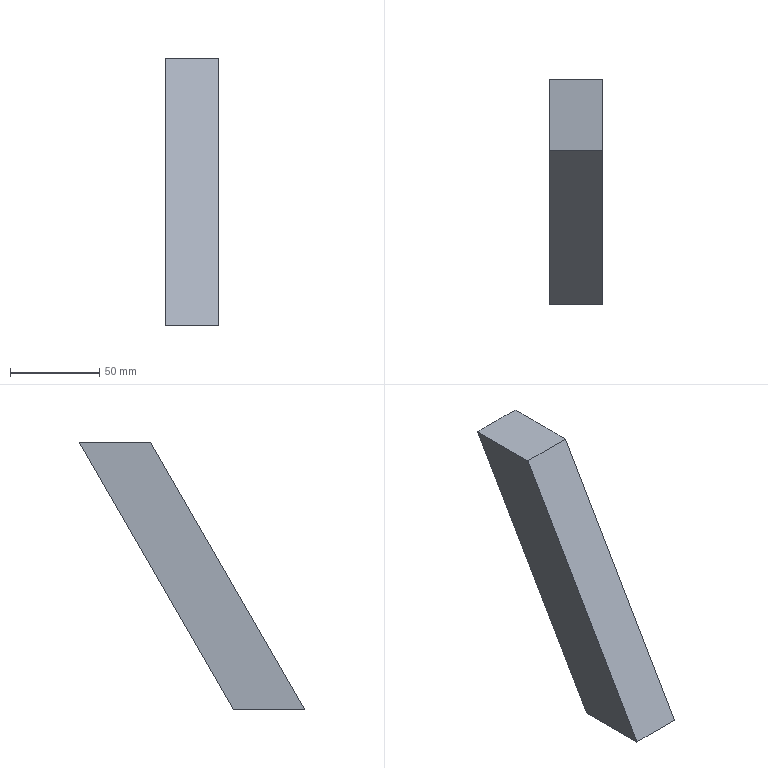Component | NX | AYAK_2 | 1 solid | 6 faces | box 30 x 126.6 x 150 mm | volume 180000 mm3 | plane 6
STEP:
#1=CARTESIAN_POINT('',(0.,0.,0.));
#2=DIRECTION('',(0.,0.,1.));
#3=DIRECTION('',(1.,0.,0.));
#4=AXIS2_PLACEMENT_3D('',#1,#2,#3);
#5=CARTESIAN_POINT('',(-1340.866,653.021,0.));
#6=VERTEX_POINT('',#5);
#7=CARTESIAN_POINT('',(-1340.866,693.021,0.));
#8=VERTEX_POINT('',#7);
#9=CARTESIAN_POINT('',(-1340.866,653.021,0.));
#10=DIRECTION('',(0.,1.,0.));
#11=VECTOR('',#10,1.);
#12=LINE('',#9,#11);
#13=CARTESIAN_POINT('',(-1310.866,653.021,0.));
#14=DIRECTION('',(0.,0.,1.));
#15=DIRECTION('',(1.,0.,0.));
#16=AXIS2_PLACEMENT_3D('',#13,#14,#15);
#17=PLANE('',#16);
#18=CARTESIAN_POINT('',(-30.,0.));
#19=DIRECTION('',(0.,1.));
#20=VECTOR('',#19,1.);
#21=LINE('',#18,#20);
#22=(GEOMETRIC_REPRESENTATION_CONTEXT(2)PARAMETRIC_REPRESENTATION_CONTEXT()REPRESENTATION_CONTEXT('',''));
#23=DEFINITIONAL_REPRESENTATION('',(#21),#22);
#24=PCURVE('',#17,#23);
#25=CARTESIAN_POINT('',(-1340.866,653.021,0.));
#26=DIRECTION('',(1.,0.,0.));
#27=DIRECTION('',(0.,0.,-1.));
#28=AXIS2_PLACEMENT_3D('',#25,#26,#27);
#29=PLANE('',#28);
#30=CARTESIAN_POINT('',(0.,0.));
#31=DIRECTION('',(0.,1.));
#32=VECTOR('',#31,1.);
#33=LINE('',#30,#32);
#34=(GEOMETRIC_REPRESENTATION_CONTEXT(2)PARAMETRIC_REPRESENTATION_CONTEXT()REPRESENTATION_CONTEXT('',''));
#35=DEFINITIONAL_REPRESENTATION('',(#33),#34);
#36=PCURVE('',#29,#35);
#37=SURFACE_CURVE('',#12,(#24,#36),.PCURVE_S1.);
#38=EDGE_CURVE('',#6,#8,#37,.T.);
#39=ORIENTED_EDGE('',*,*,#38,.T.);
#40=CARTESIAN_POINT('',(-1310.866,693.021,0.));
#41=VERTEX_POINT('',#40);
#42=CARTESIAN_POINT('',(-1310.866,693.021,0.));
#43=DIRECTION('',(-1.,0.,0.));
#44=VECTOR('',#43,1.);
#45=LINE('',#42,#44);
#46=CARTESIAN_POINT('',(0.,40.));
#47=DIRECTION('',(-1.,0.));
#48=VECTOR('',#47,1.);
#49=LINE('',#46,#48);
#50=(GEOMETRIC_REPRESENTATION_CONTEXT(2)PARAMETRIC_REPRESENTATION_CONTEXT()REPRESENTATION_CONTEXT('',''));
#51=DEFINITIONAL_REPRESENTATION('',(#49),#50);
#52=PCURVE('',#17,#51);
#53=CARTESIAN_POINT('',(-1310.866,693.021,0.));
#54=DIRECTION('',(0.,-0.866,0.5));
#55=DIRECTION('',(0.,-0.5,-0.866));
#56=AXIS2_PLACEMENT_3D('',#53,#54,#55);
#57=PLANE('',#56);
#58=CARTESIAN_POINT('',(0.,0.));
#59=DIRECTION('',(0.,-1.));
#60=VECTOR('',#59,1.);
#61=LINE('',#58,#60);
#62=(GEOMETRIC_REPRESENTATION_CONTEXT(2)PARAMETRIC_REPRESENTATION_CONTEXT()REPRESENTATION_CONTEXT('',''));
#63=DEFINITIONAL_REPRESENTATION('',(#61),#62);
#64=PCURVE('',#57,#63);
#65=SURFACE_CURVE('',#45,(#52,#64),.PCURVE_S1.);
#66=EDGE_CURVE('',#41,#8,#65,.T.);
#67=ORIENTED_EDGE('',*,*,#66,.F.);
#68=CARTESIAN_POINT('',(-1310.866,653.021,0.));
#69=VERTEX_POINT('',#68);
#70=CARTESIAN_POINT('',(-1310.866,653.021,0.));
#71=DIRECTION('',(0.,1.,0.));
#72=VECTOR('',#71,1.);
#73=LINE('',#70,#72);
#74=CARTESIAN_POINT('',(0.,0.));
#75=DIRECTION('',(0.,1.));
#76=VECTOR('',#75,1.);
#77=LINE('',#74,#76);
#78=(GEOMETRIC_REPRESENTATION_CONTEXT(2)PARAMETRIC_REPRESENTATION_CONTEXT()REPRESENTATION_CONTEXT('',''));
#79=DEFINITIONAL_REPRESENTATION('',(#77),#78);
#80=PCURVE('',#17,#79);
#81=CARTESIAN_POINT('',(-1310.866,653.021,0.));
#82=DIRECTION('',(1.,0.,0.));
#83=DIRECTION('',(0.,0.,-1.));
#84=AXIS2_PLACEMENT_3D('',#81,#82,#83);
#85=PLANE('',#84);
#86=CARTESIAN_POINT('',(0.,0.));
#87=DIRECTION('',(0.,1.));
#88=VECTOR('',#87,1.);
#89=LINE('',#86,#88);
#90=(GEOMETRIC_REPRESENTATION_CONTEXT(2)PARAMETRIC_REPRESENTATION_CONTEXT()REPRESENTATION_CONTEXT('',''));
#91=DEFINITIONAL_REPRESENTATION('',(#89),#90);
#92=PCURVE('',#85,#91);
#93=SURFACE_CURVE('',#73,(#80,#92),.PCURVE_S1.);
#94=EDGE_CURVE('',#69,#41,#93,.T.);
#95=ORIENTED_EDGE('',*,*,#94,.F.);
#96=CARTESIAN_POINT('',(-1310.866,653.021,0.));
#97=DIRECTION('',(-1.,0.,0.));
#98=VECTOR('',#97,1.);
#99=LINE('',#96,#98);
#100=CARTESIAN_POINT('',(0.,0.));
#101=DIRECTION('',(-1.,0.));
#102=VECTOR('',#101,1.);
#103=LINE('',#100,#102);
#104=(GEOMETRIC_REPRESENTATION_CONTEXT(2)PARAMETRIC_REPRESENTATION_CONTEXT()REPRESENTATION_CONTEXT('',''));
#105=DEFINITIONAL_REPRESENTATION('',(#103),#104);
#106=PCURVE('',#17,#105);
#107=CARTESIAN_POINT('',(-1310.866,739.623,150.));
#108=DIRECTION('',(0.,0.866,-0.5));
#109=DIRECTION('',(0.,0.5,0.866));
#110=AXIS2_PLACEMENT_3D('',#107,#108,#109);
#111=PLANE('',#110);
#112=CARTESIAN_POINT('',(-173.205,0.));
#113=DIRECTION('',(0.,-1.));
#114=VECTOR('',#113,1.);
#115=LINE('',#112,#114);
#116=(GEOMETRIC_REPRESENTATION_CONTEXT(2)PARAMETRIC_REPRESENTATION_CONTEXT()REPRESENTATION_CONTEXT('',''));
#117=DEFINITIONAL_REPRESENTATION('',(#115),#116);
#118=PCURVE('',#111,#117);
#119=SURFACE_CURVE('',#99,(#106,#118),.PCURVE_S1.);
#120=EDGE_CURVE('',#69,#6,#119,.T.);
#121=ORIENTED_EDGE('',*,*,#120,.T.);
#122=EDGE_LOOP('',(#39,#67,#95,#121));
#123=FACE_BOUND('',#122,.T.);
#124=ADVANCED_FACE('',(#123),#17,.F.);
#125=CARTESIAN_POINT('',(-1340.866,779.623,150.));
#126=VERTEX_POINT('',#125);
#127=CARTESIAN_POINT('',(-1340.866,693.021,0.));
#128=DIRECTION('',(0.,0.5,0.866));
#129=VECTOR('',#128,1.);
#130=LINE('',#127,#129);
#131=CARTESIAN_POINT('',(0.,-30.));
#132=DIRECTION('',(-1.,0.));
#133=VECTOR('',#132,1.);
#134=LINE('',#131,#133);
#135=(GEOMETRIC_REPRESENTATION_CONTEXT(2)PARAMETRIC_REPRESENTATION_CONTEXT()REPRESENTATION_CONTEXT('',''));
#136=DEFINITIONAL_REPRESENTATION('',(#134),#135);
#137=PCURVE('',#57,#136);
#138=CARTESIAN_POINT('',(0.,40.));
#139=DIRECTION('',(-0.866,0.5));
#140=VECTOR('',#139,1.);
#141=LINE('',#138,#140);
#142=(GEOMETRIC_REPRESENTATION_CONTEXT(2)PARAMETRIC_REPRESENTATION_CONTEXT()REPRESENTATION_CONTEXT('',''));
#143=DEFINITIONAL_REPRESENTATION('',(#141),#142);
#144=PCURVE('',#29,#143);
#145=SURFACE_CURVE('',#130,(#137,#144),.PCURVE_S1.);
#146=EDGE_CURVE('',#8,#126,#145,.T.);
#147=ORIENTED_EDGE('',*,*,#146,.T.);
#148=CARTESIAN_POINT('',(-1310.866,779.623,150.));
#149=VERTEX_POINT('',#148);
#150=CARTESIAN_POINT('',(-1310.866,779.623,150.));
#151=DIRECTION('',(-1.,0.,0.));
#152=VECTOR('',#151,1.);
#153=LINE('',#150,#152);
#154=CARTESIAN_POINT('',(-173.205,0.));
#155=DIRECTION('',(0.,-1.));
#156=VECTOR('',#155,1.);
#157=LINE('',#154,#156);
#158=(GEOMETRIC_REPRESENTATION_CONTEXT(2)PARAMETRIC_REPRESENTATION_CONTEXT()REPRESENTATION_CONTEXT('',''));
#159=DEFINITIONAL_REPRESENTATION('',(#157),#158);
#160=PCURVE('',#57,#159);
#161=CARTESIAN_POINT('',(-1310.866,779.623,150.));
#162=DIRECTION('',(0.,0.,-1.));
#163=DIRECTION('',(-1.,0.,0.));
#164=AXIS2_PLACEMENT_3D('',#161,#162,#163);
#165=PLANE('',#164);
#166=CARTESIAN_POINT('',(0.,0.));
#167=DIRECTION('',(1.,0.));
#168=VECTOR('',#167,1.);
#169=LINE('',#166,#168);
#170=(GEOMETRIC_REPRESENTATION_CONTEXT(2)PARAMETRIC_REPRESENTATION_CONTEXT()REPRESENTATION_CONTEXT('',''));
#171=DEFINITIONAL_REPRESENTATION('',(#169),#170);
#172=PCURVE('',#165,#171);
#173=SURFACE_CURVE('',#153,(#160,#172),.PCURVE_S1.);
#174=EDGE_CURVE('',#149,#126,#173,.T.);
#175=ORIENTED_EDGE('',*,*,#174,.F.);
#176=CARTESIAN_POINT('',(-1310.866,693.021,0.));
#177=DIRECTION('',(0.,0.5,0.866));
#178=VECTOR('',#177,1.);
#179=LINE('',#176,#178);
#180=CARTESIAN_POINT('',(0.,0.));
#181=DIRECTION('',(-1.,0.));
#182=VECTOR('',#181,1.);
#183=LINE('',#180,#182);
#184=(GEOMETRIC_REPRESENTATION_CONTEXT(2)PARAMETRIC_REPRESENTATION_CONTEXT()REPRESENTATION_CONTEXT('',''));
#185=DEFINITIONAL_REPRESENTATION('',(#183),#184);
#186=PCURVE('',#57,#185);
#187=CARTESIAN_POINT('',(0.,40.));
#188=DIRECTION('',(-0.866,0.5));
#189=VECTOR('',#188,1.);
#190=LINE('',#187,#189);
#191=(GEOMETRIC_REPRESENTATION_CONTEXT(2)PARAMETRIC_REPRESENTATION_CONTEXT()REPRESENTATION_CONTEXT('',''));
#192=DEFINITIONAL_REPRESENTATION('',(#190),#191);
#193=PCURVE('',#85,#192);
#194=SURFACE_CURVE('',#179,(#186,#193),.PCURVE_S1.);
#195=EDGE_CURVE('',#41,#149,#194,.T.);
#196=ORIENTED_EDGE('',*,*,#195,.F.);
#197=ORIENTED_EDGE('',*,*,#66,.T.);
#198=EDGE_LOOP('',(#147,#175,#196,#197));
#199=FACE_BOUND('',#198,.T.);
#200=ADVANCED_FACE('',(#199),#57,.F.);
#201=CARTESIAN_POINT('',(-1340.866,739.623,150.));
#202=VERTEX_POINT('',#201);
#203=CARTESIAN_POINT('',(-1340.866,779.623,150.));
#204=DIRECTION('',(0.,-1.,0.));
#205=VECTOR('',#204,1.);
#206=LINE('',#203,#205);
#207=CARTESIAN_POINT('',(30.,0.));
#208=DIRECTION('',(0.,-1.));
#209=VECTOR('',#208,1.);
#210=LINE('',#207,#209);
#211=(GEOMETRIC_REPRESENTATION_CONTEXT(2)PARAMETRIC_REPRESENTATION_CONTEXT()REPRESENTATION_CONTEXT('',''));
#212=DEFINITIONAL_REPRESENTATION('',(#210),#211);
#213=PCURVE('',#165,#212);
#214=CARTESIAN_POINT('',(-150.,126.603));
#215=DIRECTION('',(0.,-1.));
#216=VECTOR('',#215,1.);
#217=LINE('',#214,#216);
#218=(GEOMETRIC_REPRESENTATION_CONTEXT(2)PARAMETRIC_REPRESENTATION_CONTEXT()REPRESENTATION_CONTEXT('',''));
#219=DEFINITIONAL_REPRESENTATION('',(#217),#218);
#220=PCURVE('',#29,#219);
#221=SURFACE_CURVE('',#206,(#213,#220),.PCURVE_S1.);
#222=EDGE_CURVE('',#126,#202,#221,.T.);
#223=ORIENTED_EDGE('',*,*,#222,.T.);
#224=CARTESIAN_POINT('',(-1310.866,739.623,150.));
#225=VERTEX_POINT('',#224);
#226=CARTESIAN_POINT('',(-1310.866,739.623,150.));
#227=DIRECTION('',(-1.,0.,0.));
#228=VECTOR('',#227,1.);
#229=LINE('',#226,#228);
#230=CARTESIAN_POINT('',(0.,-40.));
#231=DIRECTION('',(1.,0.));
#232=VECTOR('',#231,1.);
#233=LINE('',#230,#232);
#234=(GEOMETRIC_REPRESENTATION_CONTEXT(2)PARAMETRIC_REPRESENTATION_CONTEXT()REPRESENTATION_CONTEXT('',''));
#235=DEFINITIONAL_REPRESENTATION('',(#233),#234);
#236=PCURVE('',#165,#235);
#237=CARTESIAN_POINT('',(0.,0.));
#238=DIRECTION('',(0.,-1.));
#239=VECTOR('',#238,1.);
#240=LINE('',#237,#239);
#241=(GEOMETRIC_REPRESENTATION_CONTEXT(2)PARAMETRIC_REPRESENTATION_CONTEXT()REPRESENTATION_CONTEXT('',''));
#242=DEFINITIONAL_REPRESENTATION('',(#240),#241);
#243=PCURVE('',#111,#242);
#244=SURFACE_CURVE('',#229,(#236,#243),.PCURVE_S1.);
#245=EDGE_CURVE('',#225,#202,#244,.T.);
#246=ORIENTED_EDGE('',*,*,#245,.F.);
#247=CARTESIAN_POINT('',(-1310.866,779.623,150.));
#248=DIRECTION('',(0.,-1.,0.));
#249=VECTOR('',#248,1.);
#250=LINE('',#247,#249);
#251=CARTESIAN_POINT('',(0.,0.));
#252=DIRECTION('',(0.,-1.));
#253=VECTOR('',#252,1.);
#254=LINE('',#251,#253);
#255=(GEOMETRIC_REPRESENTATION_CONTEXT(2)PARAMETRIC_REPRESENTATION_CONTEXT()REPRESENTATION_CONTEXT('',''));
#256=DEFINITIONAL_REPRESENTATION('',(#254),#255);
#257=PCURVE('',#165,#256);
#258=CARTESIAN_POINT('',(-150.,126.603));
#259=DIRECTION('',(0.,-1.));
#260=VECTOR('',#259,1.);
#261=LINE('',#258,#260);
#262=(GEOMETRIC_REPRESENTATION_CONTEXT(2)PARAMETRIC_REPRESENTATION_CONTEXT()REPRESENTATION_CONTEXT('',''));
#263=DEFINITIONAL_REPRESENTATION('',(#261),#262);
#264=PCURVE('',#85,#263);
#265=SURFACE_CURVE('',#250,(#257,#264),.PCURVE_S1.);
#266=EDGE_CURVE('',#149,#225,#265,.T.);
#267=ORIENTED_EDGE('',*,*,#266,.F.);
#268=ORIENTED_EDGE('',*,*,#174,.T.);
#269=EDGE_LOOP('',(#223,#246,#267,#268));
#270=FACE_BOUND('',#269,.T.);
#271=ADVANCED_FACE('',(#270),#165,.F.);
#272=CARTESIAN_POINT('',(-1340.866,739.623,150.));
#273=DIRECTION('',(0.,-0.5,-0.866));
#274=VECTOR('',#273,1.);
#275=LINE('',#272,#274);
#276=CARTESIAN_POINT('',(0.,-30.));
#277=DIRECTION('',(-1.,0.));
#278=VECTOR('',#277,1.);
#279=LINE('',#276,#278);
#280=(GEOMETRIC_REPRESENTATION_CONTEXT(2)PARAMETRIC_REPRESENTATION_CONTEXT()REPRESENTATION_CONTEXT('',''));
#281=DEFINITIONAL_REPRESENTATION('',(#279),#280);
#282=PCURVE('',#111,#281);
#283=CARTESIAN_POINT('',(-150.,86.603));
#284=DIRECTION('',(0.866,-0.5));
#285=VECTOR('',#284,1.);
#286=LINE('',#283,#285);
#287=(GEOMETRIC_REPRESENTATION_CONTEXT(2)PARAMETRIC_REPRESENTATION_CONTEXT()REPRESENTATION_CONTEXT('',''));
#288=DEFINITIONAL_REPRESENTATION('',(#286),#287);
#289=PCURVE('',#29,#288);
#290=SURFACE_CURVE('',#275,(#282,#289),.PCURVE_S1.);
#291=EDGE_CURVE('',#202,#6,#290,.T.);
#292=ORIENTED_EDGE('',*,*,#291,.T.);
#293=ORIENTED_EDGE('',*,*,#120,.F.);
#294=CARTESIAN_POINT('',(-1310.866,739.623,150.));
#295=DIRECTION('',(0.,-0.5,-0.866));
#296=VECTOR('',#295,1.);
#297=LINE('',#294,#296);
#298=CARTESIAN_POINT('',(0.,0.));
#299=DIRECTION('',(-1.,0.));
#300=VECTOR('',#299,1.);
#301=LINE('',#298,#300);
#302=(GEOMETRIC_REPRESENTATION_CONTEXT(2)PARAMETRIC_REPRESENTATION_CONTEXT()REPRESENTATION_CONTEXT('',''));
#303=DEFINITIONAL_REPRESENTATION('',(#301),#302);
#304=PCURVE('',#111,#303);
#305=CARTESIAN_POINT('',(-150.,86.603));
#306=DIRECTION('',(0.866,-0.5));
#307=VECTOR('',#306,1.);
#308=LINE('',#305,#307);
#309=(GEOMETRIC_REPRESENTATION_CONTEXT(2)PARAMETRIC_REPRESENTATION_CONTEXT()REPRESENTATION_CONTEXT('',''));
#310=DEFINITIONAL_REPRESENTATION('',(#308),#309);
#311=PCURVE('',#85,#310);
#312=SURFACE_CURVE('',#297,(#304,#311),.PCURVE_S1.);
#313=EDGE_CURVE('',#225,#69,#312,.T.);
#314=ORIENTED_EDGE('',*,*,#313,.F.);
#315=ORIENTED_EDGE('',*,*,#245,.T.);
#316=EDGE_LOOP('',(#292,#293,#314,#315));
#317=FACE_BOUND('',#316,.T.);
#318=ADVANCED_FACE('',(#317),#111,.F.);
#319=ORIENTED_EDGE('',*,*,#94,.T.);
#320=ORIENTED_EDGE('',*,*,#195,.T.);
#321=ORIENTED_EDGE('',*,*,#266,.T.);
#322=ORIENTED_EDGE('',*,*,#313,.T.);
#323=EDGE_LOOP('',(#319,#320,#321,#322));
#324=FACE_BOUND('',#323,.T.);
#325=ADVANCED_FACE('',(#324),#85,.T.);
#326=ORIENTED_EDGE('',*,*,#38,.F.);
#327=ORIENTED_EDGE('',*,*,#291,.F.);
#328=ORIENTED_EDGE('',*,*,#222,.F.);
#329=ORIENTED_EDGE('',*,*,#146,.F.);
#330=EDGE_LOOP('',(#326,#327,#328,#329));
#331=FACE_BOUND('',#330,.T.);
#332=ADVANCED_FACE('',(#331),#29,.F.);
#333=CLOSED_SHELL('',(#124,#200,#271,#318,#325,#332));
#334=MANIFOLD_SOLID_BREP('',#333);
#335=(LENGTH_UNIT()NAMED_UNIT(*)SI_UNIT(.MILLI.,.METRE.));
#336=UNCERTAINTY_MEASURE_WITH_UNIT(LENGTH_MEASURE(0.0000001),#335,'','');
#337=(NAMED_UNIT(*)PLANE_ANGLE_UNIT()SI_UNIT($,.RADIAN.));
#338=(NAMED_UNIT(*)SI_UNIT($,.STERADIAN.)SOLID_ANGLE_UNIT());
#339=(GEOMETRIC_REPRESENTATION_CONTEXT(3)GLOBAL_UNCERTAINTY_ASSIGNED_CONTEXT((#336))GLOBAL_UNIT_ASSIGNED_CONTEXT((#335,#337,#338))REPRESENTATION_CONTEXT('',''));
#340=ADVANCED_BREP_SHAPE_REPRESENTATION('',(#4,#334),#339);